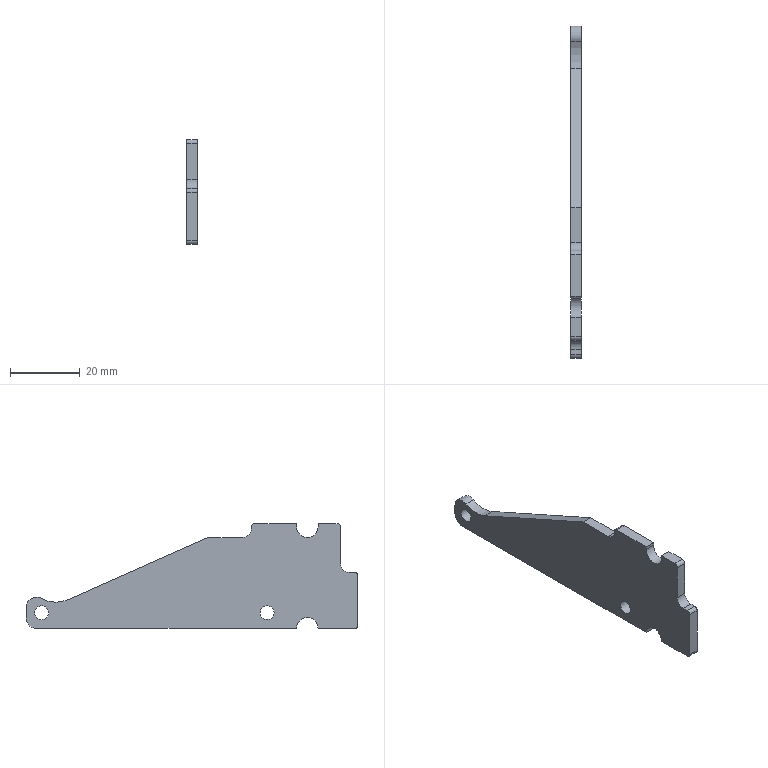Component | NX | BRACKET | 1 solid | 28 faces | volume 5669 mm3 | plane 15 | cylinder 13 | commonest cylinder face diameters 2 x4 5 x2 6.2 x2 6 x2 4 x2 17.228 x1